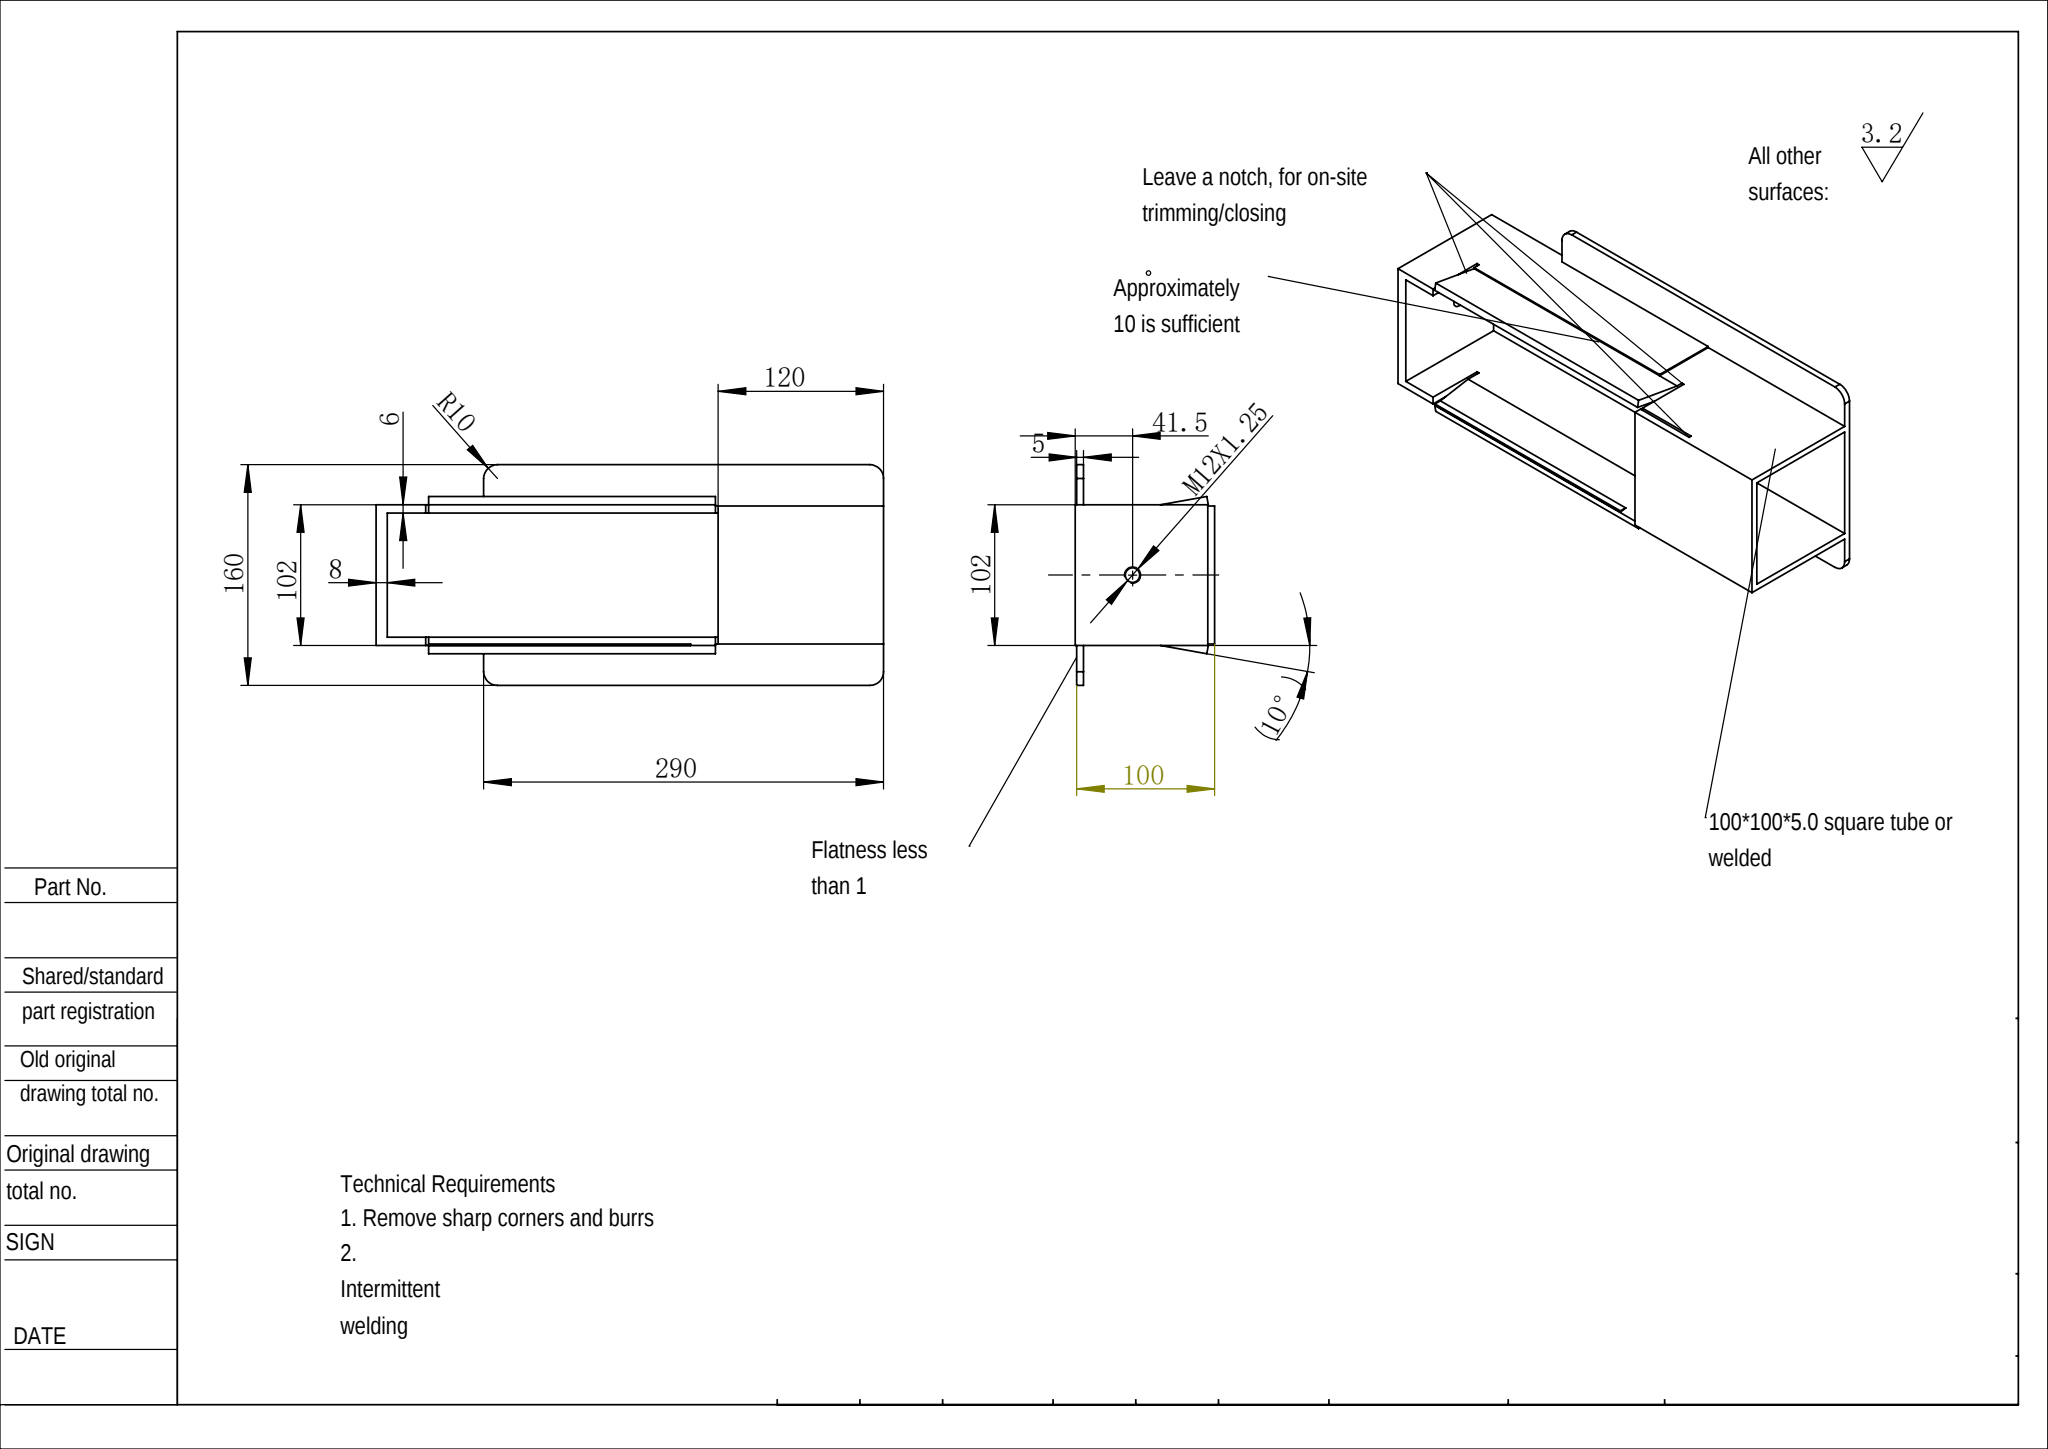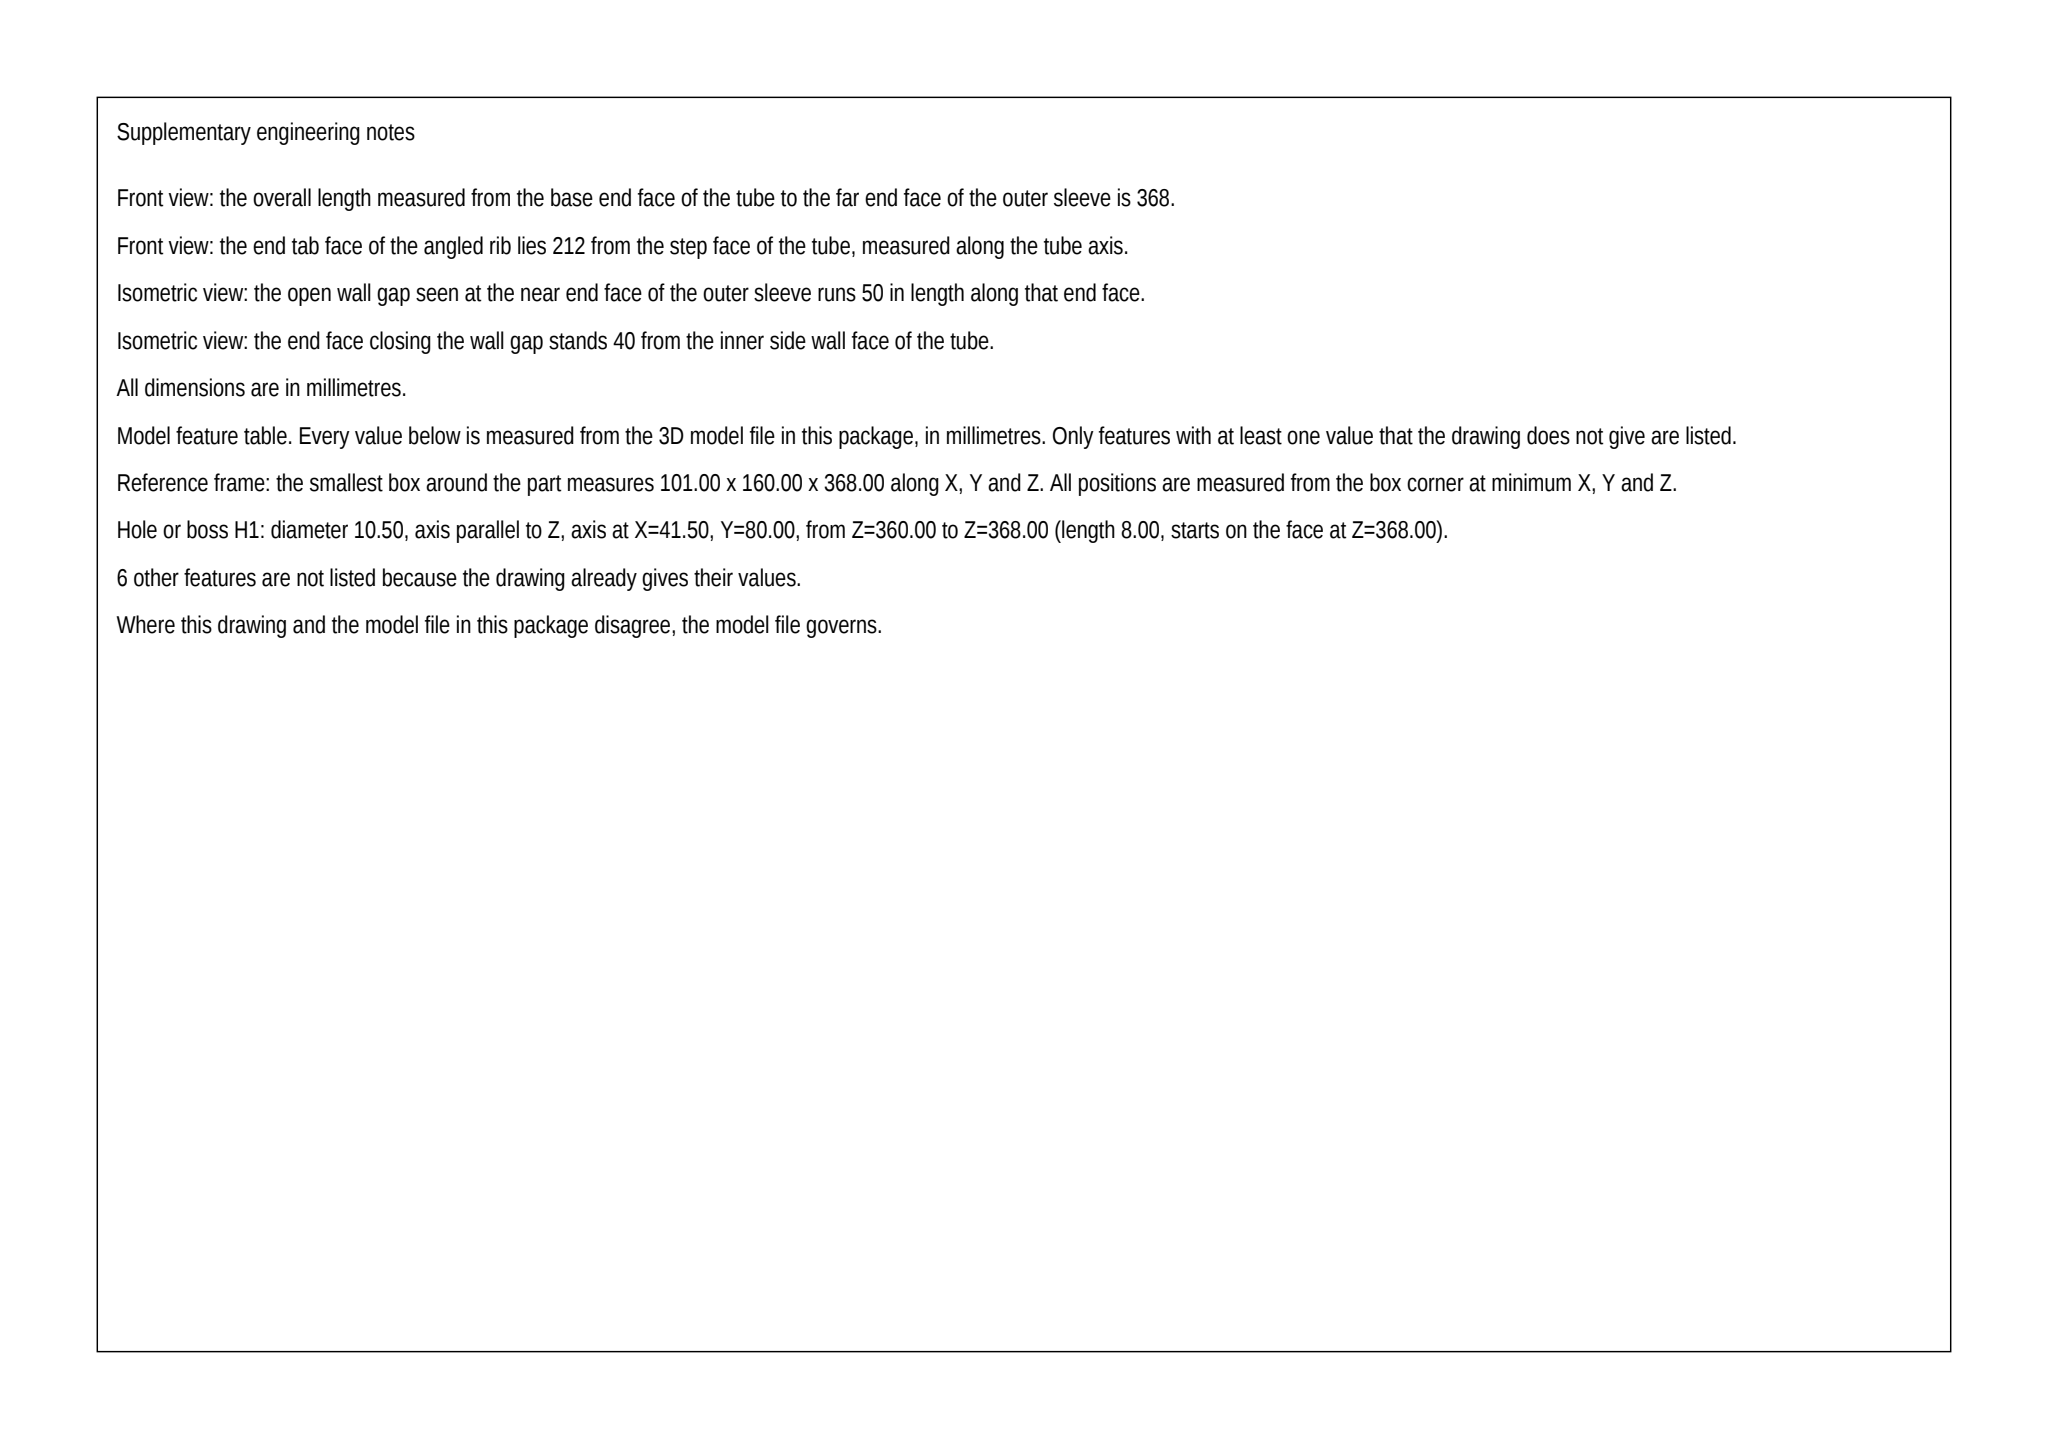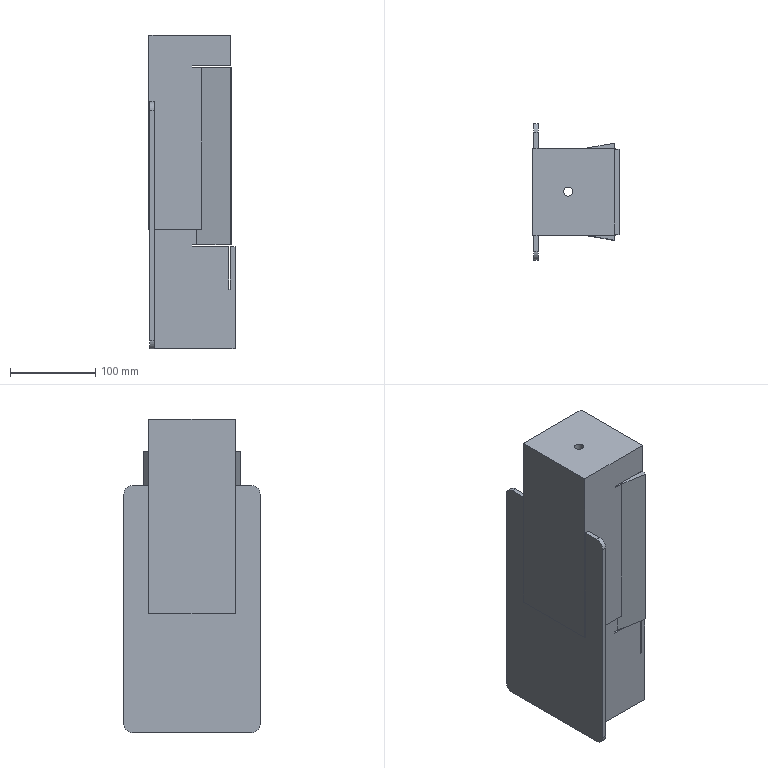Part | SolidWorks | mm | material 100*100*5.0 square tube or welded | 1 solid | 59 faces | box 101 x 160 x 368 mm | volume 790362 mm3 | plane 53 | cylinder 6 | commonest cylinder face diameters 20 x4 10.5 x2
build123d program:
from build123d import *

# Parameters (mm, degrees)
SKETCH1_W                   = 100
SKETCH1_H                   = 100
SKETCH1_W_2                 = 90
SKETCH1_H_2                 = 90
EXTRUDE_THIN1_DEPTH         = 140
EXTRUDE_THIN2_DEPTH         = 220
SKETCH7_W                   = 290
SKETCH7_H                   = 160
BOSS_EXTRUDE1_DEPTH         = 5
SKETCH8_W                   = 96
SKETCH8_H                   = 102
BOSS_EXTRUDE2_DEPTH         = 8
M12X1_25_TAPPED_HOLE1_D     = 10.5
M12X1_25_TAPPED_HOLE1_DEPTH = 22.25
M12X1_25_TAPPED_HOLE1_TIP   = 3.155
FILLET1_R                   = 10
SKETCH12_W                  = 20
SKETCH12_H                  = 100
CUT_EXTRUDE2_DEPTH          = 390.699
SKETCH13_W                  = 40
SKETCH13_H                  = 210
CUT_EXTRUDE3_DEPTH          = 632.142
BOSS_EXTRUDE3_DEPTH         = 210
SKETCH15_W                  = 2
SKETCH15_H                  = 50
CUT_EXTRUDE4_DEPTH          = 632.142
CUT_EXTRUDE5_DEPTH          = 624.43
CUT_EXTRUDE5_DEPTH_BACK     = 624.43
SKETCH17_W                  = 50
SKETCH17_H                  = 2


with BuildPart() as part:
    # Sketch1 → Extrude-Thin1 (new body)
    with BuildSketch(Plane.XY):
        with Locations((-445, -5)):
            Rectangle(SKETCH1_W, SKETCH1_H)
        with Locations((-445, -5)):
            Rectangle(SKETCH1_W_2, SKETCH1_H_2, mode=Mode.SUBTRACT)
    extrude(amount=EXTRUDE_THIN1_DEPTH)

    # Sketch3 → Extrude-Thin2 (add)
    with BuildSketch(Plane.XY.offset(140)):
        Polygon((-400, 40), (-490, 40), (-490, -50), (-400, -50), (-400, -56), (-496, -56), (-496, 46), (-400, 46), align=None)
    extrude(amount=EXTRUDE_THIN2_DEPTH)

    # Sketch7 → Boss-Extrude1 (add)
    with BuildSketch(Plane.ZY.offset(495)):
        with Locations((145, -5)):
            Rectangle(SKETCH7_W, SKETCH7_H)
    extrude(amount=-BOSS_EXTRUDE1_DEPTH)

    # Sketch8 → Boss-Extrude2 (add)
    with BuildSketch(Plane.XY.offset(360)):
        with Locations((-448, -5)):
            Rectangle(SKETCH8_W, SKETCH8_H)
    extrude(amount=BOSS_EXTRUDE2_DEPTH)

    # M12x1.25 Tapped Hole1
    with Locations(Plane.XY.offset(368)):
        with Locations((-454.5, -5)):
            Hole(M12X1_25_TAPPED_HOLE1_D / 2, depth=M12X1_25_TAPPED_HOLE1_DEPTH)
            with Locations((0, 0, -(M12X1_25_TAPPED_HOLE1_DEPTH + M12X1_25_TAPPED_HOLE1_TIP / 2))):  # 118° drill point
                Cone(0, M12X1_25_TAPPED_HOLE1_D / 2, M12X1_25_TAPPED_HOLE1_TIP, mode=Mode.SUBTRACT)

    # Fillet1
    fillet1_edges = [part.edges().sort_by_distance(p)[0] for p in [
        (-492.5, -85, 0),
        (-492.5, 75, 290),
        (-492.5, 75, 0),
        (-492.5, -85, 290),
    ]]
    fillet(fillet1_edges, radius=FILLET1_R)

    # Sketch12 → Cut-Extrude2 (cut, through all)
    with BuildSketch(Plane(origin=(-400, 0, 0), x_dir=(0, 0, -1), z_dir=(1, 0, 0))):
        with Locations((-130, -5)):
            Rectangle(SKETCH12_W, SKETCH12_H)
    extrude(amount=CUT_EXTRUDE2_DEPTH, mode=Mode.SUBTRACT)

    # Sketch13 → Cut-Extrude3 (cut, through all)
    with BuildSketch(Plane.XZ.offset(55)):
        with Locations((-420, 225)):
            Rectangle(SKETCH13_W, SKETCH13_H)
    extrude(amount=-CUT_EXTRUDE3_DEPTH, mode=Mode.SUBTRACT)

    # Sketch14 → Boss-Extrude3 (add)
    with BuildSketch(Plane.XY.offset(120)):
        Polygon((-400.608, 51.946), (-440, 45), (-405.447, 45), (-399.566, 46.037), align=None)
        Polygon((-405.447, 45), (-440, 45), (-440, 40), (-433.804, 40), align=None)
        Polygon((-405.447, -55), (-440, -55), (-400.608, -61.946), (-399.566, -56.037), align=None)
        Polygon((-433.804, -50), (-440, -50), (-440, -55), (-405.447, -55), align=None)
    extrude(amount=BOSS_EXTRUDE3_DEPTH)

    # Sketch15 → Cut-Extrude4 (cut, through all)
    with BuildSketch(Plane.XZ.offset(55)):
        with Locations((-401.608, 95)):
            Rectangle(SKETCH15_W, SKETCH15_H)
    extrude(amount=-CUT_EXTRUDE4_DEPTH, mode=Mode.SUBTRACT)

    # Sketch17 → Cut-Extrude5 (cut, two sides: drawn at the far end of the back side and taken through both)
    with BuildSketch(Plane(origin=(0, 0, 0), x_dir=(1, 0, 0), z_dir=(0, 1, 0)).offset(-CUT_EXTRUDE5_DEPTH_BACK)):
        with Locations((-420, -121)):
            Rectangle(SKETCH17_W, SKETCH17_H)
        with Locations((-420, -331)):
            Rectangle(SKETCH17_W, SKETCH17_H)
    extrude(amount=CUT_EXTRUDE5_DEPTH + CUT_EXTRUDE5_DEPTH_BACK, mode=Mode.SUBTRACT)


solid = part.part